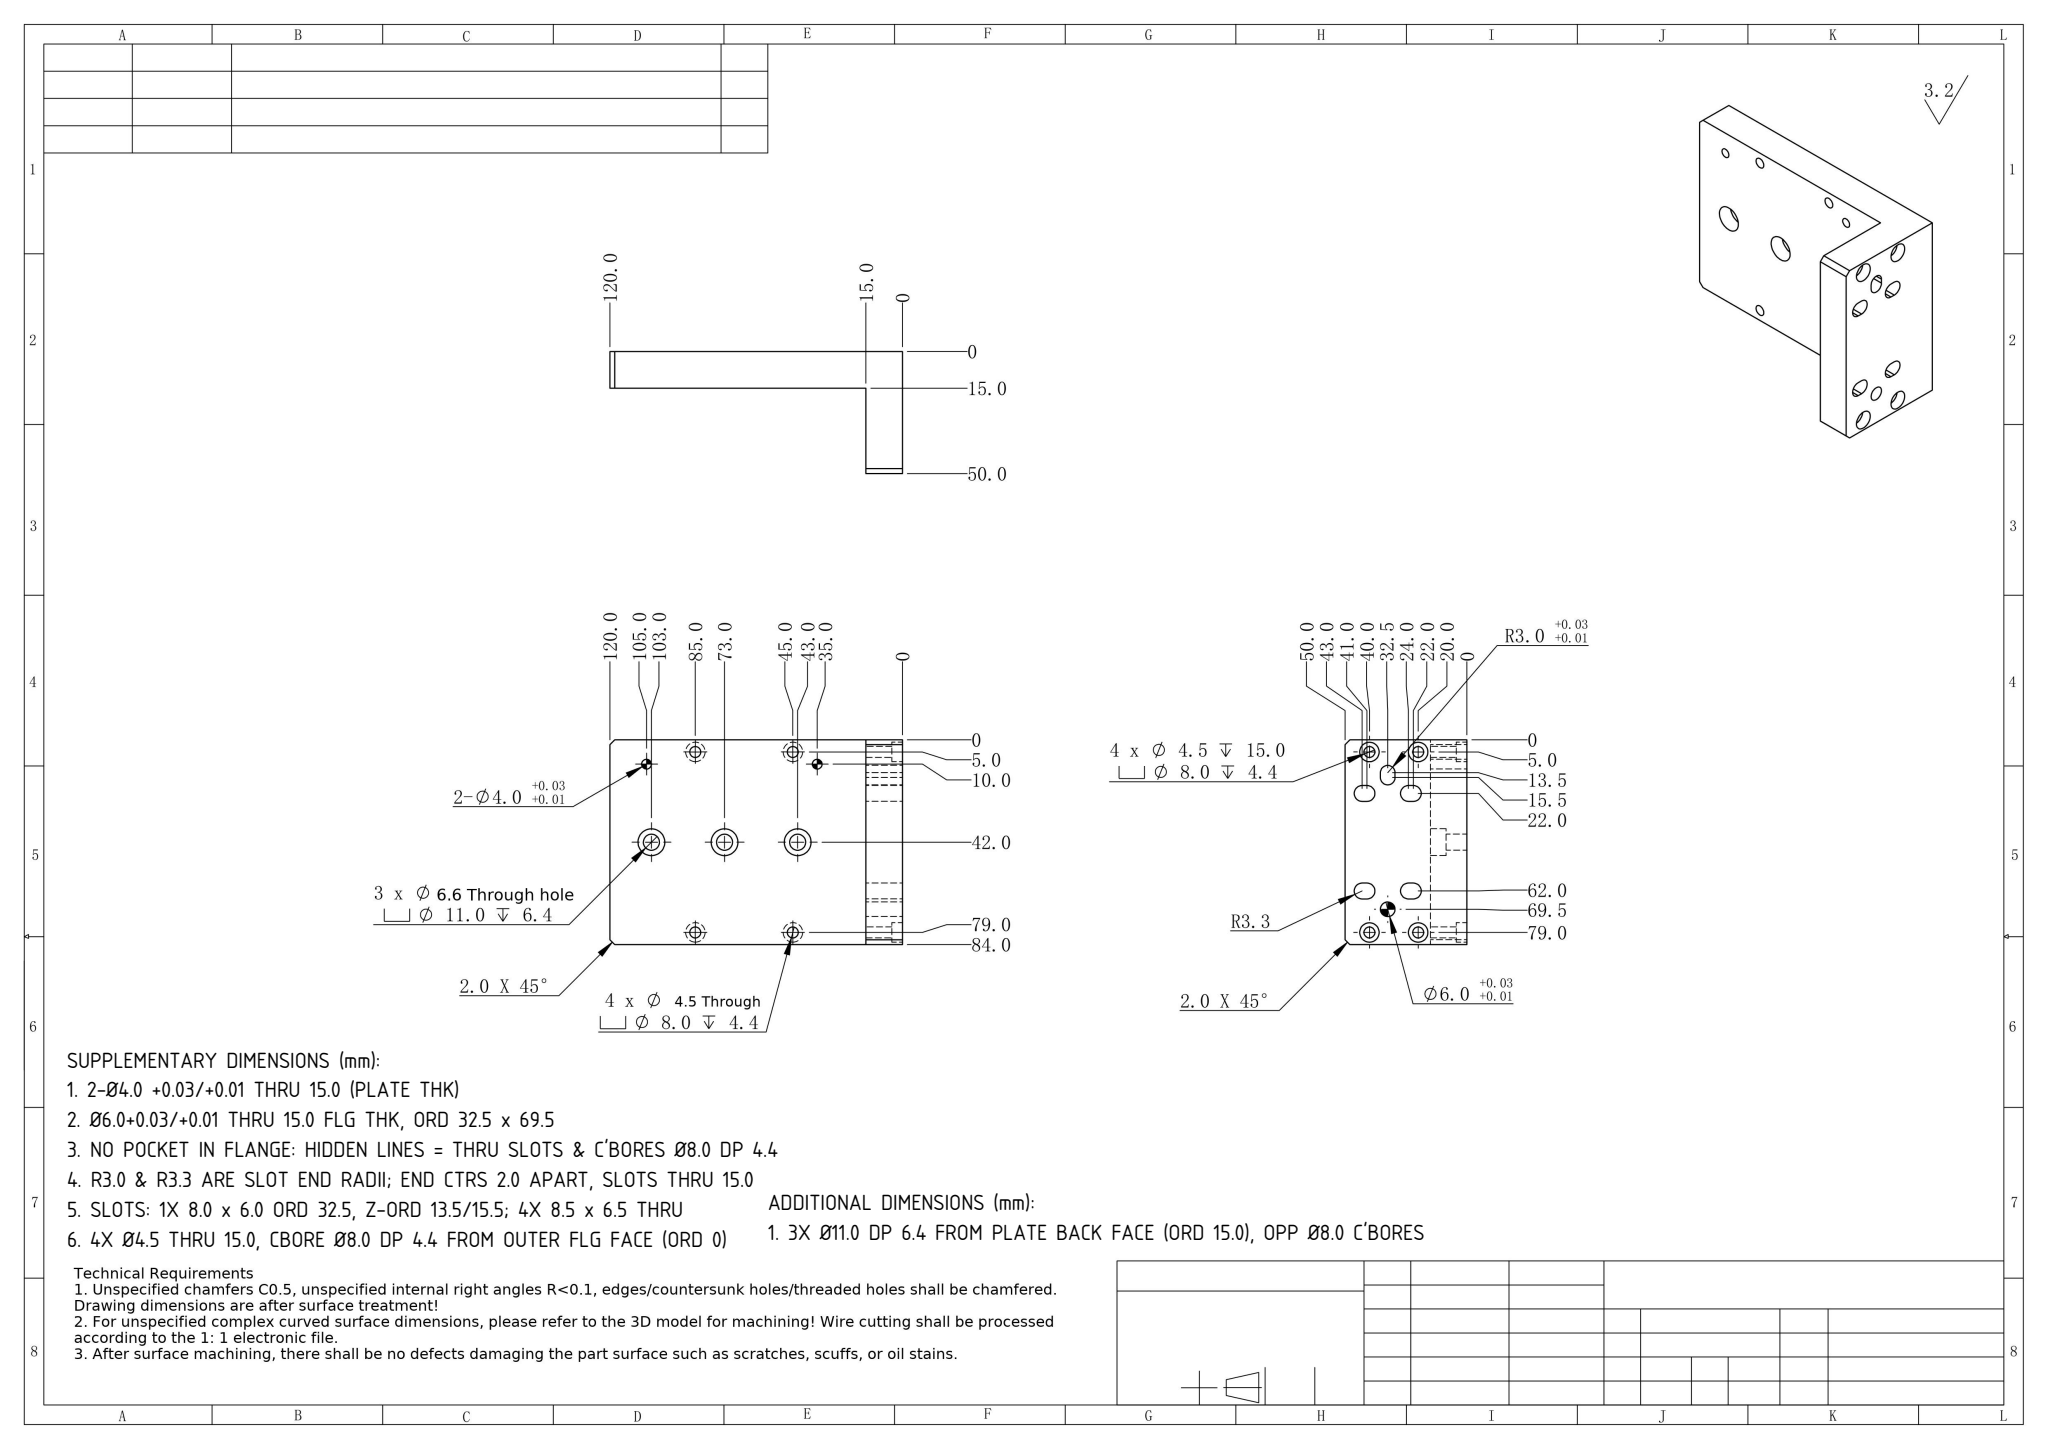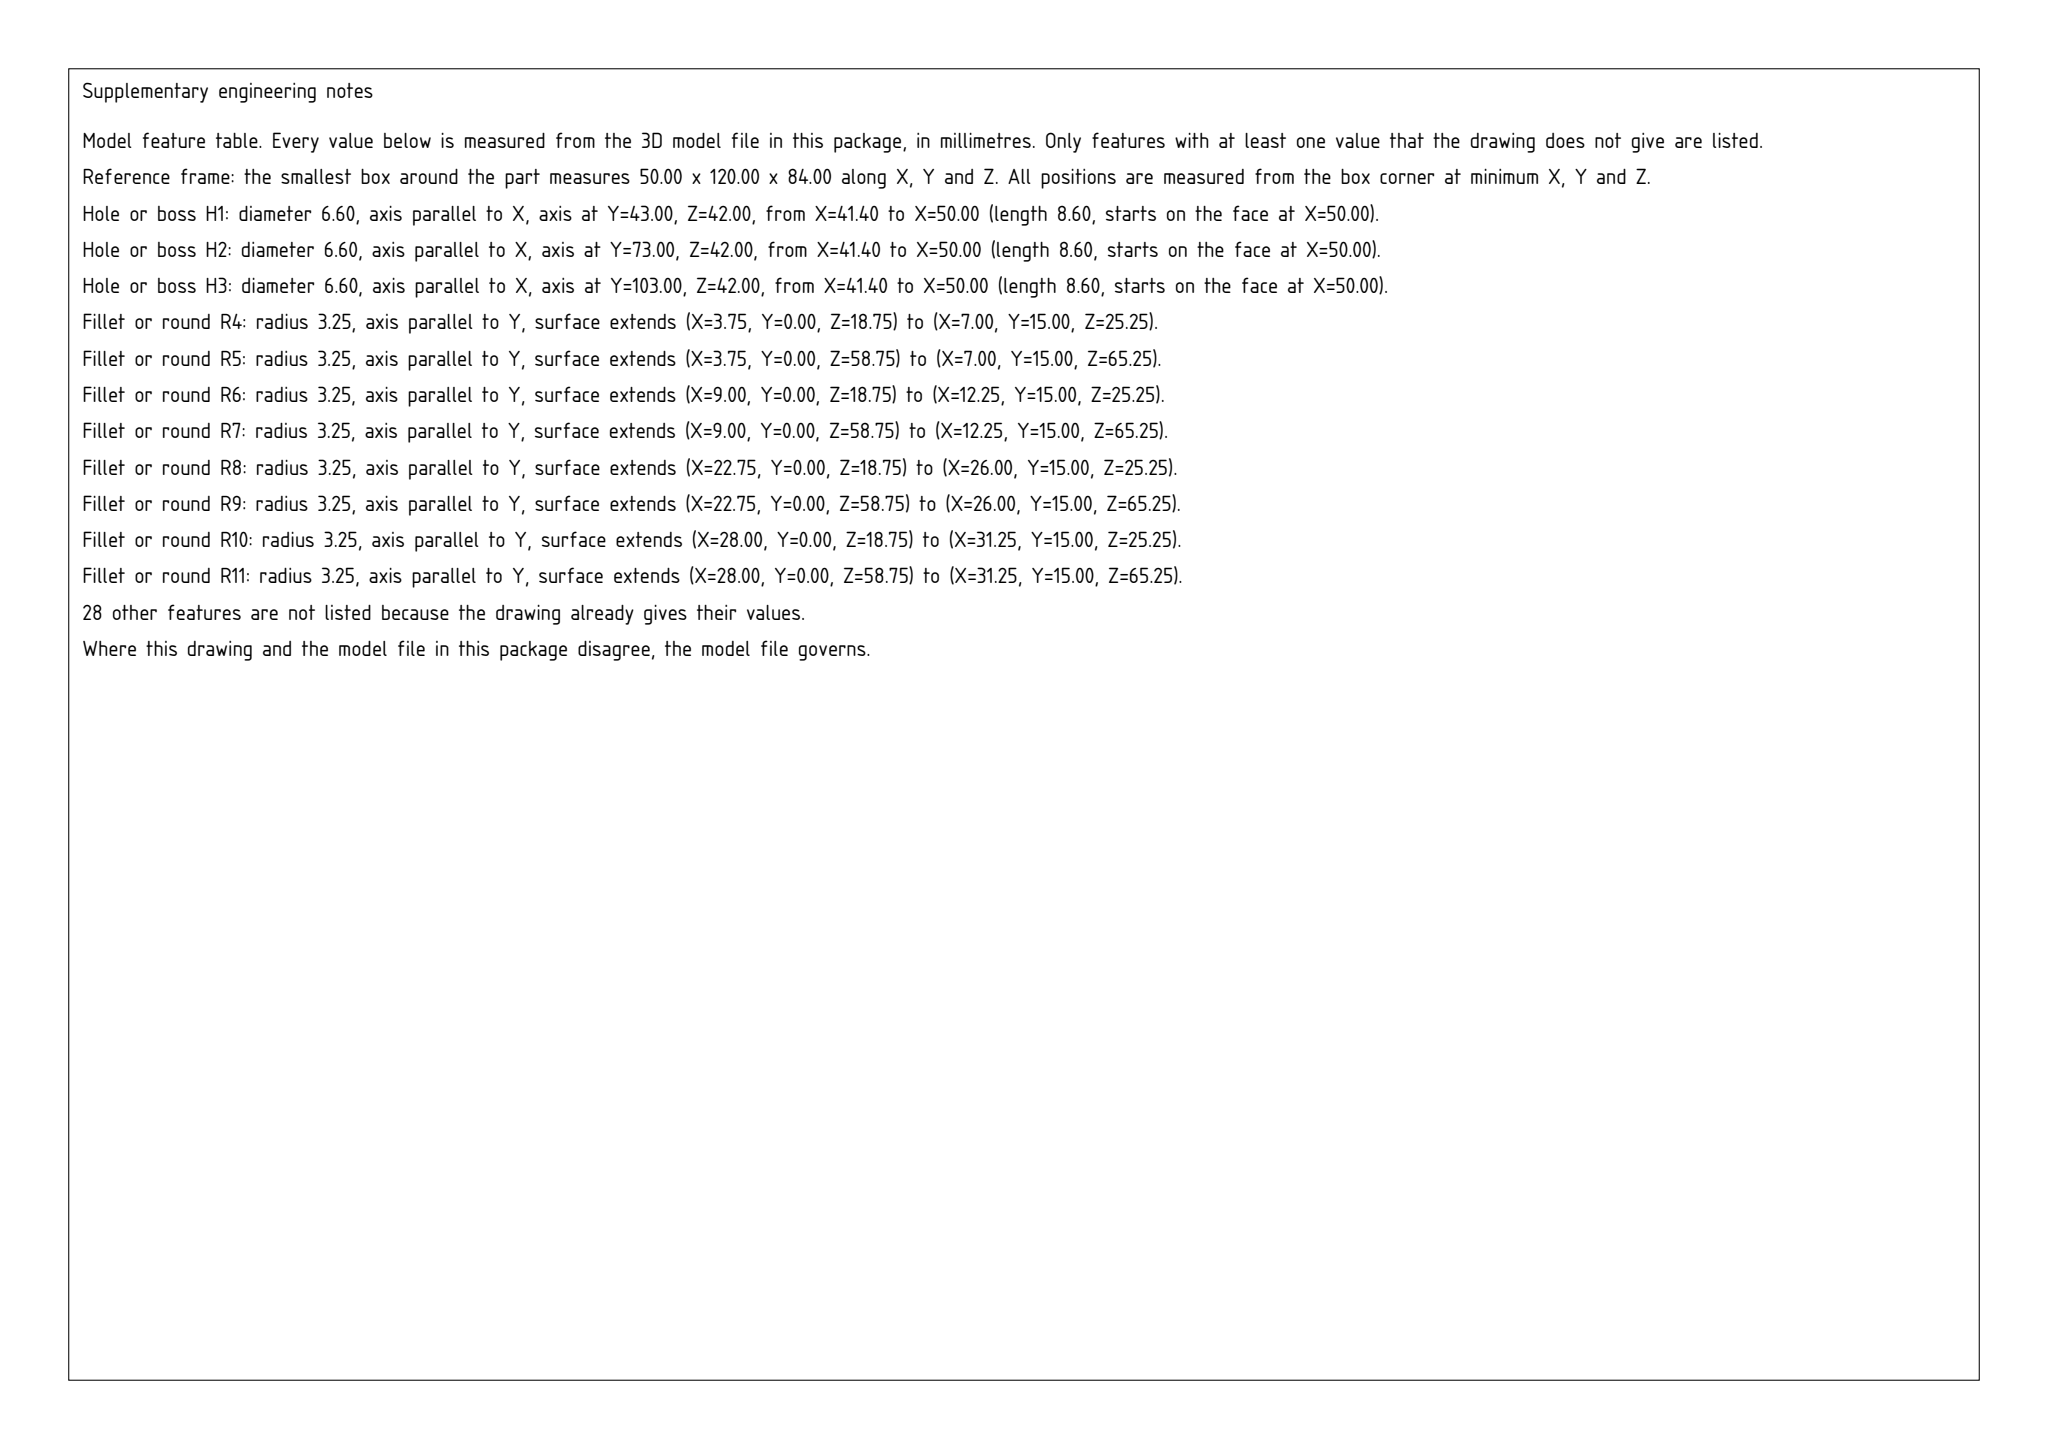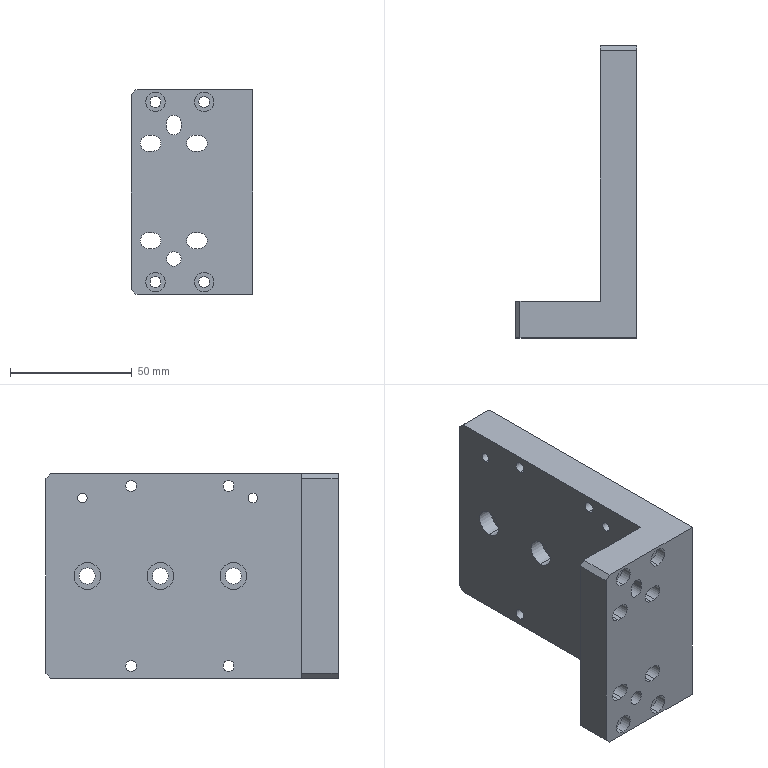Part | SolidWorks | mm | 1 solid | 97 faces | box 50 x 120 x 84 mm | volume 185178 mm3 | cylinder 64 | plane 33 | commonest cylinder face diameters 8 x16 4.5 x16 6.5 x12 11 x6 6.6 x6 6 x4 4 x4